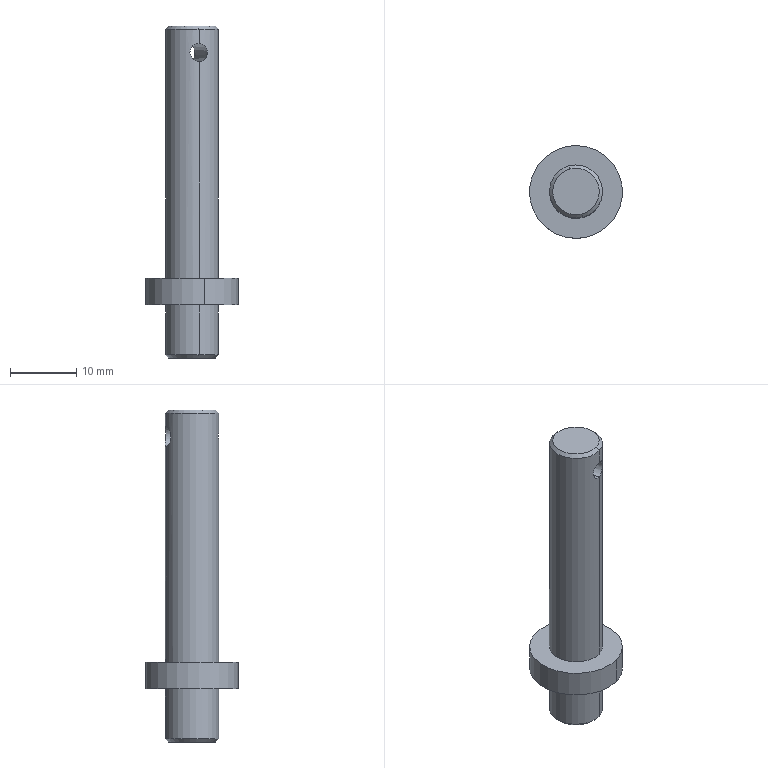Component | SolidWorks | 18Pin-1 | 1 solid | 16 faces | box 14 x 14 x 50 mm | volume 2871 mm3 | cone 6 | cylinder 6 | plane 4 | commonest cylinder face diameters 8 x4 14 x2
build123d program:
from build123d import *

# Parameters (mm, degrees)
SKETCH2_R           = 4
BOSS_EXTRUDE2_DEPTH = 50
BOSS_EXTRUDE3_START = -8
SKETCH3_R           = 7
BOSS_EXTRUDE3_DEPTH = 4
CHAMFER1_SIZE       = 0.5


with BuildPart() as part:
    # Sketch2 → Boss-Extrude2 (new body)
    with BuildSketch(Plane(origin=(0, 0, 0), x_dir=(0, 0, -1), z_dir=(1, 0, 0))):
        Circle(SKETCH2_R)
    extrude(amount=BOSS_EXTRUDE2_DEPTH)

    # Sketch3 → Boss-Extrude3 (add)
    with BuildSketch(Plane.ZY.offset(BOSS_EXTRUDE3_START)):
        Circle(SKETCH3_R)
    extrude(amount=-BOSS_EXTRUDE3_DEPTH)

    # Cut-Extrude1 cone 1 section (on through the dimple's axis) → Cut-Extrude1 (revolve, cut)
    with BuildSketch(Plane(origin=(46, 0, 4), x_dir=(0, -1, 0), z_dir=(1, 0, 0))):
        Polygon((0, 0), (1.5, 0), (0, 85.935), align=None)
    revolve(axis=Axis((46, 0, 4), (0, 0, -1)), mode=Mode.SUBTRACT)

    # Chamfer1
    chamfer1_edges = [part.edges().sort_by_distance(p)[0] for p in [
        (0, 0, 4),
        (50, 0, 4),
    ]]
    chamfer(chamfer1_edges, length=CHAMFER1_SIZE)


solid = part.part

# Placed as in the assembly
solid = solid.moved(Location((33.957, 1.776, 391), (-90, -15.475, -90)))
STEP:
#1=COLOUR_RGB('',0.7922,0.8196,0.9333);
#2=FILL_AREA_STYLE_COLOUR('',#1);
#3=FILL_AREA_STYLE('',(#2));
#4=SURFACE_STYLE_FILL_AREA(#3);
#5=SURFACE_SIDE_STYLE('',(#4));
#6=SURFACE_STYLE_USAGE(.BOTH.,#5);
#7=PRESENTATION_STYLE_ASSIGNMENT((#6));
#8=CARTESIAN_POINT('',(1.374,-0.06288,17.362));
#9=VERTEX_POINT('',#8);
#10=CARTESIAN_POINT('',(1.3,0.2027,17.362));
#11=VERTEX_POINT('',#10);
#12=CARTESIAN_POINT('',(1.337,0.06992,17.362));
#13=DIRECTION('',(-0.,-0.,1.));
#14=DIRECTION('',(0.2668,-0.9637,0.));
#15=AXIS2_PLACEMENT_3D('',#12,#13,#14);
#16=CIRCLE('',#15,0.1378);
#17=EDGE_CURVE('',#9,#11,#16,.T.);
#18=ORIENTED_EDGE('',*,*,#17,.F.);
#19=CARTESIAN_POINT('',(1.379,-0.08185,17.343));
#20=VERTEX_POINT('',#19);
#21=CARTESIAN_POINT('',(1.374,-0.06288,17.362));
#22=DIRECTION('',(0.1887,-0.6815,-0.7071));
#23=VECTOR('',#22,39.37);
#24=LINE('',#21,#23);
#25=EDGE_CURVE('',#9,#20,#24,.T.);
#26=ORIENTED_EDGE('',*,*,#25,.T.);
#27=CARTESIAN_POINT('',(1.295,0.2217,17.343));
#28=VERTEX_POINT('',#27);
#29=CARTESIAN_POINT('',(1.337,0.06992,17.343));
#30=DIRECTION('',(0.,0.,-1.));
#31=DIRECTION('',(0.2668,-0.9637,0.));
#32=AXIS2_PLACEMENT_3D('',#29,#30,#31);
#33=CIRCLE('',#32,0.1575);
#34=EDGE_CURVE('',#28,#20,#33,.T.);
#35=ORIENTED_EDGE('',*,*,#34,.F.);
#36=CARTESIAN_POINT('',(1.3,0.2027,17.362));
#37=DIRECTION('',(-0.1887,0.6815,-0.7071));
#38=VECTOR('',#37,39.37);
#39=LINE('',#36,#38);
#40=EDGE_CURVE('',#11,#28,#39,.T.);
#41=ORIENTED_EDGE('',*,*,#40,.F.);
#42=EDGE_LOOP('',(#18,#26,#35,#41));
#43=FACE_OUTER_BOUND('',#42,.T.);
#44=CARTESIAN_POINT('',(1.337,0.06992,17.362));
#45=DIRECTION('',(0.,0.,-1.));
#46=DIRECTION('',(-0.2668,0.9637,0.));
#47=AXIS2_PLACEMENT_3D('',#44,#45,#46);
#48=CONICAL_SURFACE('',#47,0.1378,0.7854);
#49=ADVANCED_FACE('',(#43),#48,.T.);
#50=CARTESIAN_POINT('',(1.3,0.2027,15.394));
#51=VERTEX_POINT('',#50);
#52=CARTESIAN_POINT('',(1.374,-0.06288,15.394));
#53=VERTEX_POINT('',#52);
#54=CARTESIAN_POINT('',(1.337,0.06992,15.394));
#55=DIRECTION('',(0.,0.,-1.));
#56=DIRECTION('',(0.2668,-0.9637,0.));
#57=AXIS2_PLACEMENT_3D('',#54,#55,#56);
#58=CIRCLE('',#57,0.1378);
#59=EDGE_CURVE('',#51,#53,#58,.T.);
#60=ORIENTED_EDGE('',*,*,#59,.F.);
#61=CARTESIAN_POINT('',(1.295,0.2217,15.413));
#62=VERTEX_POINT('',#61);
#63=CARTESIAN_POINT('',(1.295,0.2217,15.413));
#64=DIRECTION('',(-0.1887,0.6815,0.7071));
#65=VECTOR('',#64,39.37);
#66=LINE('',#63,#65);
#67=EDGE_CURVE('',#51,#62,#66,.T.);
#68=ORIENTED_EDGE('',*,*,#67,.T.);
#69=CARTESIAN_POINT('',(1.379,-0.08185,15.413));
#70=VERTEX_POINT('',#69);
#71=CARTESIAN_POINT('',(1.337,0.06992,15.413));
#72=DIRECTION('',(-0.,-0.,1.));
#73=DIRECTION('',(0.2668,-0.9637,0.));
#74=AXIS2_PLACEMENT_3D('',#71,#72,#73);
#75=CIRCLE('',#74,0.1575);
#76=EDGE_CURVE('',#70,#62,#75,.T.);
#77=ORIENTED_EDGE('',*,*,#76,.F.);
#78=CARTESIAN_POINT('',(1.379,-0.08185,15.413));
#79=DIRECTION('',(0.1887,-0.6815,0.7071));
#80=VECTOR('',#79,39.37);
#81=LINE('',#78,#80);
#82=EDGE_CURVE('',#53,#70,#81,.T.);
#83=ORIENTED_EDGE('',*,*,#82,.F.);
#84=EDGE_LOOP('',(#60,#68,#77,#83));
#85=FACE_OUTER_BOUND('',#84,.T.);
#86=CARTESIAN_POINT('',(1.337,0.06992,15.413));
#87=DIRECTION('',(-0.,-0.,1.));
#88=DIRECTION('',(0.2668,-0.9637,0.));
#89=AXIS2_PLACEMENT_3D('',#86,#87,#88);
#90=CONICAL_SURFACE('',#89,0.1575,0.7854);
#91=ADVANCED_FACE('',(#85),#90,.T.);
#92=CARTESIAN_POINT('',(1.379,-0.08185,17.151));
#93=VERTEX_POINT('',#92);
#94=CARTESIAN_POINT('',(1.379,-0.08185,17.258));
#95=VERTEX_POINT('',#94);
#96=CARTESIAN_POINT('',(1.379,-0.08185,17.151));
#97=CARTESIAN_POINT('',(1.372,-0.08373,17.151));
#98=CARTESIAN_POINT('',(1.365,-0.08514,17.153));
#99=CARTESIAN_POINT('',(1.355,-0.0865,17.157));
#100=CARTESIAN_POINT('',(1.352,-0.08683,17.158));
#101=CARTESIAN_POINT('',(1.346,-0.0873,17.162));
#102=CARTESIAN_POINT('',(1.344,-0.08743,17.164));
#103=CARTESIAN_POINT('',(1.336,-0.08764,17.172));
#104=CARTESIAN_POINT('',(1.332,-0.0875,17.178));
#105=CARTESIAN_POINT('',(1.328,-0.08729,17.187));
#106=CARTESIAN_POINT('',(1.326,-0.08721,17.191));
#107=CARTESIAN_POINT('',(1.325,-0.08711,17.198));
#108=CARTESIAN_POINT('',(1.325,-0.08708,17.201));
#109=CARTESIAN_POINT('',(1.325,-0.08708,17.208));
#110=CARTESIAN_POINT('',(1.325,-0.08711,17.212));
#111=CARTESIAN_POINT('',(1.326,-0.08721,17.219));
#112=CARTESIAN_POINT('',(1.328,-0.08729,17.222));
#113=CARTESIAN_POINT('',(1.332,-0.0875,17.232));
#114=CARTESIAN_POINT('',(1.336,-0.08764,17.238));
#115=CARTESIAN_POINT('',(1.346,-0.08737,17.248));
#116=CARTESIAN_POINT('',(1.352,-0.08695,17.251));
#117=CARTESIAN_POINT('',(1.362,-0.08559,17.256));
#118=CARTESIAN_POINT('',(1.365,-0.08501,17.257));
#119=CARTESIAN_POINT('',(1.372,-0.08362,17.258));
#120=CARTESIAN_POINT('',(1.375,-0.0828,17.258));
#121=CARTESIAN_POINT('',(1.379,-0.08185,17.258));
#122=B_SPLINE_CURVE_WITH_KNOTS('',3,(#96,#97,#98,#99,#100,#101,#102,#103,#104,#105,#106,#107,#108,#109,#110,#111,#112,#113,#114,#115,#116,#117,#118,#119,#120,#121),.UNSPECIFIED.,.F.,.F.,(4,2,2,2,2,2,2,2,2,2,2,2,4),(0.007428,0.007965,0.008234,0.008502,0.009039,0.009307,0.009575,0.009844,0.01011,0.01065,0.01119,0.01145,0.01172),.UNSPECIFIED.);
#123=EDGE_CURVE('',#93,#95,#122,.T.);
#124=ORIENTED_EDGE('',*,*,#123,.F.);
#125=CARTESIAN_POINT('',(1.295,0.2217,17.146));
#126=VERTEX_POINT('',#125);
#127=CARTESIAN_POINT('',(1.295,0.2217,17.146));
#128=DIRECTION('',(-0.2668,0.9636,-0.01745));
#129=VECTOR('',#128,39.37);
#130=LINE('',#127,#129);
#131=EDGE_CURVE('',#93,#126,#130,.T.);
#132=ORIENTED_EDGE('',*,*,#131,.T.);
#133=CARTESIAN_POINT('',(1.295,0.2217,17.264));
#134=VERTEX_POINT('',#133);
#135=CARTESIAN_POINT('',(1.295,0.2217,17.264));
#136=CARTESIAN_POINT('',(1.291,0.2206,17.264));
#137=CARTESIAN_POINT('',(1.287,0.2195,17.263));
#138=CARTESIAN_POINT('',(1.28,0.2169,17.262));
#139=CARTESIAN_POINT('',(1.277,0.2155,17.261));
#140=CARTESIAN_POINT('',(1.267,0.2112,17.256));
#141=CARTESIAN_POINT('',(1.261,0.208,17.252));
#142=CARTESIAN_POINT('',(1.251,0.2023,17.241));
#143=CARTESIAN_POINT('',(1.248,0.1997,17.235));
#144=CARTESIAN_POINT('',(1.244,0.197,17.224));
#145=CARTESIAN_POINT('',(1.243,0.1962,17.22));
#146=CARTESIAN_POINT('',(1.242,0.1952,17.212));
#147=CARTESIAN_POINT('',(1.241,0.195,17.209));
#148=CARTESIAN_POINT('',(1.241,0.195,17.201));
#149=CARTESIAN_POINT('',(1.242,0.1952,17.197));
#150=CARTESIAN_POINT('',(1.243,0.1962,17.189));
#151=CARTESIAN_POINT('',(1.244,0.197,17.186));
#152=CARTESIAN_POINT('',(1.246,0.1988,17.178));
#153=CARTESIAN_POINT('',(1.248,0.1999,17.175));
#154=CARTESIAN_POINT('',(1.252,0.2024,17.169));
#155=CARTESIAN_POINT('',(1.254,0.2038,17.166));
#156=CARTESIAN_POINT('',(1.259,0.2066,17.16));
#157=CARTESIAN_POINT('',(1.261,0.2081,17.158));
#158=CARTESIAN_POINT('',(1.267,0.2111,17.154));
#159=CARTESIAN_POINT('',(1.27,0.2126,17.152));
#160=CARTESIAN_POINT('',(1.28,0.217,17.147));
#161=CARTESIAN_POINT('',(1.287,0.2196,17.146));
#162=CARTESIAN_POINT('',(1.295,0.2217,17.146));
#163=B_SPLINE_CURVE_WITH_KNOTS('',3,(#135,#136,#137,#138,#139,#140,#141,#142,#143,#144,#145,#146,#147,#148,#149,#150,#151,#152,#153,#154,#155,#156,#157,#158,#159,#160,#161,#162),.UNSPECIFIED.,.F.,.F.,(4,2,2,2,2,2,2,2,2,2,2,2,2,4),(0.005986,0.006282,0.006577,0.007167,0.007758,0.008053,0.008348,0.008643,0.008939,0.009234,0.009529,0.009824,0.01012,0.01071),.UNSPECIFIED.);
#164=EDGE_CURVE('',#134,#126,#163,.T.);
#165=ORIENTED_EDGE('',*,*,#164,.F.);
#166=CARTESIAN_POINT('',(1.295,0.2217,17.264));
#167=DIRECTION('',(-0.2668,0.9636,0.01745));
#168=VECTOR('',#167,39.37);
#169=LINE('',#166,#168);
#170=EDGE_CURVE('',#95,#134,#169,.T.);
#171=ORIENTED_EDGE('',*,*,#170,.F.);
#172=EDGE_LOOP('',(#124,#132,#165,#171));
#173=FACE_OUTER_BOUND('',#172,.T.);
#174=CARTESIAN_POINT('',(1.295,0.2217,17.205));
#175=DIRECTION('',(-0.2668,0.9637,-0.));
#176=DIRECTION('',(0.,0.,1.));
#177=AXIS2_PLACEMENT_3D('',#174,#175,#176);
#178=CONICAL_SURFACE('',#177,0.05906,0.01745);
#179=ADVANCED_FACE('',(#173),#178,.F.);
#180=CARTESIAN_POINT('',(1.295,0.2217,15.709));
#181=VERTEX_POINT('',#180);
#182=CARTESIAN_POINT('',(1.379,-0.08185,15.709));
#183=VERTEX_POINT('',#182);
#184=CARTESIAN_POINT('',(1.337,0.06992,15.709));
#185=DIRECTION('',(0.,0.,-1.));
#186=DIRECTION('',(-0.2668,0.9637,0.));
#187=AXIS2_PLACEMENT_3D('',#184,#185,#186);
#188=CIRCLE('',#187,0.1575);
#189=EDGE_CURVE('',#181,#183,#188,.T.);
#190=ORIENTED_EDGE('',*,*,#189,.T.);
#191=CARTESIAN_POINT('',(1.379,-0.08185,17.362));
#192=DIRECTION('',(0.,0.,-1.));
#193=VECTOR('',#192,39.37);
#194=LINE('',#191,#193);
#195=EDGE_CURVE('',#183,#70,#194,.T.);
#196=ORIENTED_EDGE('',*,*,#195,.T.);
#197=ORIENTED_EDGE('',*,*,#76,.T.);
#198=CARTESIAN_POINT('',(1.295,0.2217,17.362));
#199=DIRECTION('',(0.,0.,-1.));
#200=VECTOR('',#199,39.37);
#201=LINE('',#198,#200);
#202=EDGE_CURVE('',#181,#62,#201,.T.);
#203=ORIENTED_EDGE('',*,*,#202,.F.);
#204=EDGE_LOOP('',(#190,#196,#197,#203));
#205=FACE_OUTER_BOUND('',#204,.T.);
#206=CARTESIAN_POINT('',(1.337,0.06992,17.362));
#207=DIRECTION('',(0.,0.,-1.));
#208=DIRECTION('',(-0.2668,0.9637,0.));
#209=AXIS2_PLACEMENT_3D('',#206,#207,#208);
#210=CYLINDRICAL_SURFACE('',#209,0.1575);
#211=ADVANCED_FACE('',(#205),#210,.T.);
#212=CARTESIAN_POINT('',(1.263,0.3355,15.866));
#213=VERTEX_POINT('',#212);
#214=CARTESIAN_POINT('',(1.41,-0.1957,15.866));
#215=VERTEX_POINT('',#214);
#216=CARTESIAN_POINT('',(1.337,0.06992,15.866));
#217=DIRECTION('',(0.,0.,-1.));
#218=DIRECTION('',(-0.2668,0.9637,0.));
#219=AXIS2_PLACEMENT_3D('',#216,#217,#218);
#220=CIRCLE('',#219,0.2756);
#221=EDGE_CURVE('',#213,#215,#220,.T.);
#222=ORIENTED_EDGE('',*,*,#221,.T.);
#223=CARTESIAN_POINT('',(1.41,-0.1957,15.709));
#224=VERTEX_POINT('',#223);
#225=CARTESIAN_POINT('',(1.41,-0.1957,15.866));
#226=DIRECTION('',(0.,0.,-1.));
#227=VECTOR('',#226,39.37);
#228=LINE('',#225,#227);
#229=EDGE_CURVE('',#215,#224,#228,.T.);
#230=ORIENTED_EDGE('',*,*,#229,.T.);
#231=CARTESIAN_POINT('',(1.263,0.3355,15.709));
#232=VERTEX_POINT('',#231);
#233=CARTESIAN_POINT('',(1.337,0.06992,15.709));
#234=DIRECTION('',(0.,0.,-1.));
#235=DIRECTION('',(-0.2668,0.9637,0.));
#236=AXIS2_PLACEMENT_3D('',#233,#234,#235);
#237=CIRCLE('',#236,0.2756);
#238=EDGE_CURVE('',#232,#224,#237,.T.);
#239=ORIENTED_EDGE('',*,*,#238,.F.);
#240=CARTESIAN_POINT('',(1.263,0.3355,15.866));
#241=DIRECTION('',(0.,0.,-1.));
#242=VECTOR('',#241,39.37);
#243=LINE('',#240,#242);
#244=EDGE_CURVE('',#213,#232,#243,.T.);
#245=ORIENTED_EDGE('',*,*,#244,.F.);
#246=EDGE_LOOP('',(#222,#230,#239,#245));
#247=FACE_OUTER_BOUND('',#246,.T.);
#248=CARTESIAN_POINT('',(1.337,0.06992,15.866));
#249=DIRECTION('',(0.,0.,-1.));
#250=DIRECTION('',(-0.2668,0.9637,0.));
#251=AXIS2_PLACEMENT_3D('',#248,#249,#250);
#252=CYLINDRICAL_SURFACE('',#251,0.2756);
#253=ADVANCED_FACE('',(#247),#252,.T.);
#254=ORIENTED_EDGE('',*,*,#34,.T.);
#255=CARTESIAN_POINT('',(1.379,-0.08185,17.362));
#256=DIRECTION('',(0.,0.,-1.));
#257=VECTOR('',#256,39.37);
#258=LINE('',#255,#257);
#259=EDGE_CURVE('',#20,#95,#258,.T.);
#260=ORIENTED_EDGE('',*,*,#259,.T.);
#261=CARTESIAN_POINT('',(1.379,-0.08185,17.258));
#262=CARTESIAN_POINT('',(1.386,-0.07995,17.258));
#263=CARTESIAN_POINT('',(1.392,-0.07759,17.257));
#264=CARTESIAN_POINT('',(1.404,-0.07246,17.251));
#265=CARTESIAN_POINT('',(1.41,-0.06972,17.247));
#266=CARTESIAN_POINT('',(1.419,-0.06474,17.238));
#267=CARTESIAN_POINT('',(1.422,-0.06248,17.232));
#268=CARTESIAN_POINT('',(1.427,-0.05932,17.219));
#269=CARTESIAN_POINT('',(1.428,-0.05841,17.212));
#270=CARTESIAN_POINT('',(1.428,-0.05841,17.201));
#271=CARTESIAN_POINT('',(1.428,-0.05863,17.198));
#272=CARTESIAN_POINT('',(1.427,-0.05948,17.191));
#273=CARTESIAN_POINT('',(1.426,-0.0601,17.187));
#274=CARTESIAN_POINT('',(1.422,-0.06249,17.178));
#275=CARTESIAN_POINT('',(1.419,-0.06475,17.172));
#276=CARTESIAN_POINT('',(1.412,-0.06851,17.164));
#277=CARTESIAN_POINT('',(1.41,-0.0698,17.162));
#278=CARTESIAN_POINT('',(1.404,-0.07243,17.158));
#279=CARTESIAN_POINT('',(1.401,-0.07377,17.157));
#280=CARTESIAN_POINT('',(1.392,-0.07759,17.153));
#281=CARTESIAN_POINT('',(1.386,-0.07997,17.151));
#282=CARTESIAN_POINT('',(1.379,-0.08185,17.151));
#283=B_SPLINE_CURVE_WITH_KNOTS('',3,(#261,#262,#263,#264,#265,#266,#267,#268,#269,#270,#271,#272,#273,#274,#275,#276,#277,#278,#279,#280,#281,#282),.UNSPECIFIED.,.F.,.F.,(4,2,2,2,2,2,2,2,2,2,4),(0.003136,0.003673,0.004209,0.004746,0.005282,0.005551,0.005819,0.006355,0.006624,0.006892,0.007428),.UNSPECIFIED.);
#284=EDGE_CURVE('',#95,#93,#283,.T.);
#285=ORIENTED_EDGE('',*,*,#284,.T.);
#286=CARTESIAN_POINT('',(1.379,-0.08185,15.866));
#287=VERTEX_POINT('',#286);
#288=CARTESIAN_POINT('',(1.379,-0.08185,17.362));
#289=DIRECTION('',(0.,0.,-1.));
#290=VECTOR('',#289,39.37);
#291=LINE('',#288,#290);
#292=EDGE_CURVE('',#93,#287,#291,.T.);
#293=ORIENTED_EDGE('',*,*,#292,.T.);
#294=CARTESIAN_POINT('',(1.295,0.2217,15.866));
#295=VERTEX_POINT('',#294);
#296=CARTESIAN_POINT('',(1.337,0.06992,15.866));
#297=DIRECTION('',(0.,0.,-1.));
#298=DIRECTION('',(-0.2668,0.9637,0.));
#299=AXIS2_PLACEMENT_3D('',#296,#297,#298);
#300=CIRCLE('',#299,0.1575);
#301=EDGE_CURVE('',#295,#287,#300,.T.);
#302=ORIENTED_EDGE('',*,*,#301,.F.);
#303=CARTESIAN_POINT('',(1.295,0.2217,17.362));
#304=DIRECTION('',(0.,0.,-1.));
#305=VECTOR('',#304,39.37);
#306=LINE('',#303,#305);
#307=EDGE_CURVE('',#126,#295,#306,.T.);
#308=ORIENTED_EDGE('',*,*,#307,.F.);
#309=CARTESIAN_POINT('',(1.295,0.2217,17.146));
#310=CARTESIAN_POINT('',(1.302,0.2238,17.146));
#311=CARTESIAN_POINT('',(1.31,0.2253,17.147));
#312=CARTESIAN_POINT('',(1.321,0.2266,17.152));
#313=CARTESIAN_POINT('',(1.324,0.2269,17.154));
#314=CARTESIAN_POINT('',(1.331,0.2273,17.158));
#315=CARTESIAN_POINT('',(1.334,0.2274,17.16));
#316=CARTESIAN_POINT('',(1.342,0.2274,17.168));
#317=CARTESIAN_POINT('',(1.347,0.2271,17.175));
#318=CARTESIAN_POINT('',(1.351,0.2267,17.186));
#319=CARTESIAN_POINT('',(1.353,0.2266,17.189));
#320=CARTESIAN_POINT('',(1.354,0.2264,17.197));
#321=CARTESIAN_POINT('',(1.355,0.2264,17.201));
#322=CARTESIAN_POINT('',(1.355,0.2264,17.213));
#323=CARTESIAN_POINT('',(1.353,0.2266,17.22));
#324=CARTESIAN_POINT('',(1.347,0.2271,17.235));
#325=CARTESIAN_POINT('',(1.342,0.2274,17.241));
#326=CARTESIAN_POINT('',(1.334,0.2274,17.249));
#327=CARTESIAN_POINT('',(1.331,0.2273,17.252));
#328=CARTESIAN_POINT('',(1.324,0.2269,17.256));
#329=CARTESIAN_POINT('',(1.321,0.2266,17.258));
#330=CARTESIAN_POINT('',(1.31,0.2253,17.262));
#331=CARTESIAN_POINT('',(1.302,0.2238,17.264));
#332=CARTESIAN_POINT('',(1.295,0.2217,17.264));
#333=B_SPLINE_CURVE_WITH_KNOTS('',3,(#309,#310,#311,#312,#313,#314,#315,#316,#317,#318,#319,#320,#321,#322,#323,#324,#325,#326,#327,#328,#329,#330,#331,#332),.UNSPECIFIED.,.F.,.F.,(4,2,2,2,2,2,2,2,2,2,2,4),(0.001261,0.001852,0.002147,0.002443,0.003033,0.003329,0.003624,0.004214,0.004805,0.0051,0.005396,0.005986),.UNSPECIFIED.);
#334=EDGE_CURVE('',#126,#134,#333,.T.);
#335=ORIENTED_EDGE('',*,*,#334,.T.);
#336=CARTESIAN_POINT('',(1.295,0.2217,17.362));
#337=DIRECTION('',(0.,0.,-1.));
#338=VECTOR('',#337,39.37);
#339=LINE('',#336,#338);
#340=EDGE_CURVE('',#28,#134,#339,.T.);
#341=ORIENTED_EDGE('',*,*,#340,.F.);
#342=EDGE_LOOP('',(#254,#260,#285,#293,#302,#308,#335,#341));
#343=FACE_OUTER_BOUND('',#342,.T.);
#344=CARTESIAN_POINT('',(1.337,0.06992,17.362));
#345=DIRECTION('',(0.,0.,-1.));
#346=DIRECTION('',(-0.2668,0.9637,0.));
#347=AXIS2_PLACEMENT_3D('',#344,#345,#346);
#348=CYLINDRICAL_SURFACE('',#347,0.1575);
#349=ADVANCED_FACE('',(#343),#348,.T.);
#350=ORIENTED_EDGE('',*,*,#259,.F.);
#351=CARTESIAN_POINT('',(1.337,0.06992,17.343));
#352=DIRECTION('',(0.,0.,-1.));
#353=DIRECTION('',(0.2668,-0.9637,0.));
#354=AXIS2_PLACEMENT_3D('',#351,#352,#353);
#355=CIRCLE('',#354,0.1575);
#356=EDGE_CURVE('',#20,#28,#355,.T.);
#357=ORIENTED_EDGE('',*,*,#356,.T.);
#358=ORIENTED_EDGE('',*,*,#340,.T.);
#359=ORIENTED_EDGE('',*,*,#164,.T.);
#360=ORIENTED_EDGE('',*,*,#307,.T.);
#361=CARTESIAN_POINT('',(1.337,0.06992,15.866));
#362=DIRECTION('',(0.,0.,-1.));
#363=DIRECTION('',(-0.2668,0.9637,0.));
#364=AXIS2_PLACEMENT_3D('',#361,#362,#363);
#365=CIRCLE('',#364,0.1575);
#366=EDGE_CURVE('',#287,#295,#365,.T.);
#367=ORIENTED_EDGE('',*,*,#366,.F.);
#368=ORIENTED_EDGE('',*,*,#292,.F.);
#369=ORIENTED_EDGE('',*,*,#123,.T.);
#370=EDGE_LOOP('',(#350,#357,#358,#359,#360,#367,#368,#369));
#371=FACE_OUTER_BOUND('',#370,.T.);
#372=CARTESIAN_POINT('',(1.337,0.06992,17.362));
#373=DIRECTION('',(0.,0.,-1.));
#374=DIRECTION('',(-0.2668,0.9637,0.));
#375=AXIS2_PLACEMENT_3D('',#372,#373,#374);
#376=CYLINDRICAL_SURFACE('',#375,0.1575);
#377=ADVANCED_FACE('',(#371),#376,.T.);
#378=CARTESIAN_POINT('',(1.337,0.06992,17.362));
#379=DIRECTION('',(-0.,-0.,1.));
#380=DIRECTION('',(0.2668,-0.9637,0.));
#381=AXIS2_PLACEMENT_3D('',#378,#379,#380);
#382=CIRCLE('',#381,0.1378);
#383=EDGE_CURVE('',#11,#9,#382,.T.);
#384=ORIENTED_EDGE('',*,*,#383,.T.);
#385=ORIENTED_EDGE('',*,*,#17,.T.);
#386=EDGE_LOOP('',(#384,#385));
#387=FACE_OUTER_BOUND('',#386,.T.);
#388=CARTESIAN_POINT('',(1.337,0.06992,17.362));
#389=DIRECTION('',(-0.,-0.,1.));
#390=DIRECTION('',(0.2668,-0.9637,0.));
#391=AXIS2_PLACEMENT_3D('',#388,#389,#390);
#392=PLANE('',#391);
#393=ADVANCED_FACE('',(#387),#392,.T.);
#394=ORIENTED_EDGE('',*,*,#229,.F.);
#395=CARTESIAN_POINT('',(1.337,0.06992,15.866));
#396=DIRECTION('',(0.,0.,-1.));
#397=DIRECTION('',(-0.2668,0.9637,0.));
#398=AXIS2_PLACEMENT_3D('',#395,#396,#397);
#399=CIRCLE('',#398,0.2756);
#400=EDGE_CURVE('',#215,#213,#399,.T.);
#401=ORIENTED_EDGE('',*,*,#400,.T.);
#402=ORIENTED_EDGE('',*,*,#244,.T.);
#403=CARTESIAN_POINT('',(1.337,0.06992,15.709));
#404=DIRECTION('',(0.,0.,-1.));
#405=DIRECTION('',(-0.2668,0.9637,0.));
#406=AXIS2_PLACEMENT_3D('',#403,#404,#405);
#407=CIRCLE('',#406,0.2756);
#408=EDGE_CURVE('',#224,#232,#407,.T.);
#409=ORIENTED_EDGE('',*,*,#408,.F.);
#410=EDGE_LOOP('',(#394,#401,#402,#409));
#411=FACE_OUTER_BOUND('',#410,.T.);
#412=CARTESIAN_POINT('',(1.337,0.06992,15.866));
#413=DIRECTION('',(0.,0.,-1.));
#414=DIRECTION('',(-0.2668,0.9637,0.));
#415=AXIS2_PLACEMENT_3D('',#412,#413,#414);
#416=CYLINDRICAL_SURFACE('',#415,0.2756);
#417=ADVANCED_FACE('',(#411),#416,.T.);
#418=ORIENTED_EDGE('',*,*,#301,.T.);
#419=ORIENTED_EDGE('',*,*,#366,.T.);
#420=EDGE_LOOP('',(#418,#419));
#421=FACE_BOUND('',#420,.T.);
#422=ORIENTED_EDGE('',*,*,#221,.F.);
#423=ORIENTED_EDGE('',*,*,#400,.F.);
#424=EDGE_LOOP('',(#422,#423));
#425=FACE_OUTER_BOUND('',#424,.T.);
#426=CARTESIAN_POINT('',(1.337,0.06992,15.866));
#427=DIRECTION('',(0.,0.,-1.));
#428=DIRECTION('',(-0.2668,0.9637,-0.));
#429=AXIS2_PLACEMENT_3D('',#426,#427,#428);
#430=PLANE('',#429);
#431=ADVANCED_FACE('',(#421,#425),#430,.F.);
#432=ORIENTED_EDGE('',*,*,#189,.F.);
#433=CARTESIAN_POINT('',(1.337,0.06992,15.709));
#434=DIRECTION('',(0.,0.,-1.));
#435=DIRECTION('',(-0.2668,0.9637,0.));
#436=AXIS2_PLACEMENT_3D('',#433,#434,#435);
#437=CIRCLE('',#436,0.1575);
#438=EDGE_CURVE('',#183,#181,#437,.T.);
#439=ORIENTED_EDGE('',*,*,#438,.F.);
#440=EDGE_LOOP('',(#432,#439));
#441=FACE_BOUND('',#440,.T.);
#442=ORIENTED_EDGE('',*,*,#238,.T.);
#443=ORIENTED_EDGE('',*,*,#408,.T.);
#444=EDGE_LOOP('',(#442,#443));
#445=FACE_OUTER_BOUND('',#444,.T.);
#446=CARTESIAN_POINT('',(1.337,0.06992,15.709));
#447=DIRECTION('',(0.,0.,-1.));
#448=DIRECTION('',(-0.2668,0.9637,-0.));
#449=AXIS2_PLACEMENT_3D('',#446,#447,#448);
#450=PLANE('',#449);
#451=ADVANCED_FACE('',(#441,#445),#450,.T.);
#452=CARTESIAN_POINT('',(1.337,0.06992,15.394));
#453=DIRECTION('',(0.,0.,-1.));
#454=DIRECTION('',(0.2668,-0.9637,0.));
#455=AXIS2_PLACEMENT_3D('',#452,#453,#454);
#456=CIRCLE('',#455,0.1378);
#457=EDGE_CURVE('',#53,#51,#456,.T.);
#458=ORIENTED_EDGE('',*,*,#457,.T.);
#459=ORIENTED_EDGE('',*,*,#59,.T.);
#460=EDGE_LOOP('',(#458,#459));
#461=FACE_OUTER_BOUND('',#460,.T.);
#462=CARTESIAN_POINT('',(1.337,0.06992,15.394));
#463=DIRECTION('',(-0.,-0.,1.));
#464=DIRECTION('',(0.2668,-0.9637,0.));
#465=AXIS2_PLACEMENT_3D('',#462,#463,#464);
#466=PLANE('',#465);
#467=ADVANCED_FACE('',(#461),#466,.F.);
#468=ORIENTED_EDGE('',*,*,#195,.F.);
#469=ORIENTED_EDGE('',*,*,#438,.T.);
#470=ORIENTED_EDGE('',*,*,#202,.T.);
#471=CARTESIAN_POINT('',(1.337,0.06992,15.413));
#472=DIRECTION('',(-0.,-0.,1.));
#473=DIRECTION('',(0.2668,-0.9637,0.));
#474=AXIS2_PLACEMENT_3D('',#471,#472,#473);
#475=CIRCLE('',#474,0.1575);
#476=EDGE_CURVE('',#62,#70,#475,.T.);
#477=ORIENTED_EDGE('',*,*,#476,.T.);
#478=EDGE_LOOP('',(#468,#469,#470,#477));
#479=FACE_OUTER_BOUND('',#478,.T.);
#480=CARTESIAN_POINT('',(1.337,0.06992,17.362));
#481=DIRECTION('',(0.,0.,-1.));
#482=DIRECTION('',(-0.2668,0.9637,0.));
#483=AXIS2_PLACEMENT_3D('',#480,#481,#482);
#484=CYLINDRICAL_SURFACE('',#483,0.1575);
#485=ADVANCED_FACE('',(#479),#484,.T.);
#486=ORIENTED_EDGE('',*,*,#131,.F.);
#487=ORIENTED_EDGE('',*,*,#284,.F.);
#488=ORIENTED_EDGE('',*,*,#170,.T.);
#489=ORIENTED_EDGE('',*,*,#334,.F.);
#490=EDGE_LOOP('',(#486,#487,#488,#489));
#491=FACE_OUTER_BOUND('',#490,.T.);
#492=CARTESIAN_POINT('',(1.295,0.2217,17.205));
#493=DIRECTION('',(-0.2668,0.9637,-0.));
#494=DIRECTION('',(0.,0.,1.));
#495=AXIS2_PLACEMENT_3D('',#492,#493,#494);
#496=CONICAL_SURFACE('',#495,0.05906,0.01745);
#497=ADVANCED_FACE('',(#491),#496,.F.);
#498=ORIENTED_EDGE('',*,*,#67,.F.);
#499=ORIENTED_EDGE('',*,*,#457,.F.);
#500=ORIENTED_EDGE('',*,*,#82,.T.);
#501=ORIENTED_EDGE('',*,*,#476,.F.);
#502=EDGE_LOOP('',(#498,#499,#500,#501));
#503=FACE_OUTER_BOUND('',#502,.T.);
#504=CARTESIAN_POINT('',(1.337,0.06992,15.413));
#505=DIRECTION('',(-0.,-0.,1.));
#506=DIRECTION('',(0.2668,-0.9637,0.));
#507=AXIS2_PLACEMENT_3D('',#504,#505,#506);
#508=CONICAL_SURFACE('',#507,0.1575,0.7854);
#509=ADVANCED_FACE('',(#503),#508,.T.);
#510=ORIENTED_EDGE('',*,*,#25,.F.);
#511=ORIENTED_EDGE('',*,*,#383,.F.);
#512=ORIENTED_EDGE('',*,*,#40,.T.);
#513=ORIENTED_EDGE('',*,*,#356,.F.);
#514=EDGE_LOOP('',(#510,#511,#512,#513));
#515=FACE_OUTER_BOUND('',#514,.T.);
#516=CARTESIAN_POINT('',(1.337,0.06992,17.362));
#517=DIRECTION('',(0.,0.,-1.));
#518=DIRECTION('',(-0.2668,0.9637,0.));
#519=AXIS2_PLACEMENT_3D('',#516,#517,#518);
#520=CONICAL_SURFACE('',#519,0.1378,0.7854);
#521=ADVANCED_FACE('',(#515),#520,.T.);
#522=CLOSED_SHELL('',(#49,#91,#179,#211,#253,#349,#377,#393,#417,#431,#451,#467,#485,#497,#509,#521));
#523=MANIFOLD_SOLID_BREP('',#522);
#524=STYLED_ITEM('',(#7),#523);
#525=PRESENTATION_LAYER_ASSIGNMENT('','',(#524));
#526=CARTESIAN_POINT('',(0.,0.,0.));
#527=DIRECTION('',(0.,0.,1.));
#528=DIRECTION('',(1.,0.,0.));
#529=AXIS2_PLACEMENT_3D('',#526,#527,#528);
#530=(LENGTH_UNIT()NAMED_UNIT(*)SI_UNIT($,.METRE.));
#531=LENGTH_MEASURE_WITH_UNIT(LENGTH_MEASURE(0.0254),#530);
#532=DIMENSIONAL_EXPONENTS(1.,0.,0.,0.,0.,0.,0.);
#533=(CONVERSION_BASED_UNIT('',#531)LENGTH_UNIT()NAMED_UNIT(#532));
#534=UNCERTAINTY_MEASURE_WITH_UNIT(LENGTH_MEASURE(0.00001),#533,'','');
#535=(NAMED_UNIT(*)PLANE_ANGLE_UNIT()SI_UNIT($,.RADIAN.));
#536=(NAMED_UNIT(*)SI_UNIT($,.STERADIAN.)SOLID_ANGLE_UNIT());
#537=(GEOMETRIC_REPRESENTATION_CONTEXT(3)GLOBAL_UNCERTAINTY_ASSIGNED_CONTEXT((#534))GLOBAL_UNIT_ASSIGNED_CONTEXT((#533,#535,#536))REPRESENTATION_CONTEXT('',''));
#538=ADVANCED_BREP_SHAPE_REPRESENTATION('',(#523,#529),#537);
#539=(LENGTH_UNIT()NAMED_UNIT(*)SI_UNIT($,.METRE.));
#540=LENGTH_MEASURE_WITH_UNIT(LENGTH_MEASURE(0.0254),#539);
#541=DIMENSIONAL_EXPONENTS(1.,0.,0.,0.,0.,0.,0.);
#542=(CONVERSION_BASED_UNIT('',#540)LENGTH_UNIT()NAMED_UNIT(#541));
#543=UNCERTAINTY_MEASURE_WITH_UNIT(LENGTH_MEASURE(0.00001),#542,'','');
#544=(NAMED_UNIT(*)PLANE_ANGLE_UNIT()SI_UNIT($,.RADIAN.));
#545=(NAMED_UNIT(*)SI_UNIT($,.STERADIAN.)SOLID_ANGLE_UNIT());
#546=(GEOMETRIC_REPRESENTATION_CONTEXT(3)GLOBAL_UNCERTAINTY_ASSIGNED_CONTEXT((#543))GLOBAL_UNIT_ASSIGNED_CONTEXT((#542,#544,#545))REPRESENTATION_CONTEXT('',''));
#547=MECHANICAL_DESIGN_GEOMETRIC_PRESENTATION_REPRESENTATION('',(#524),#546);